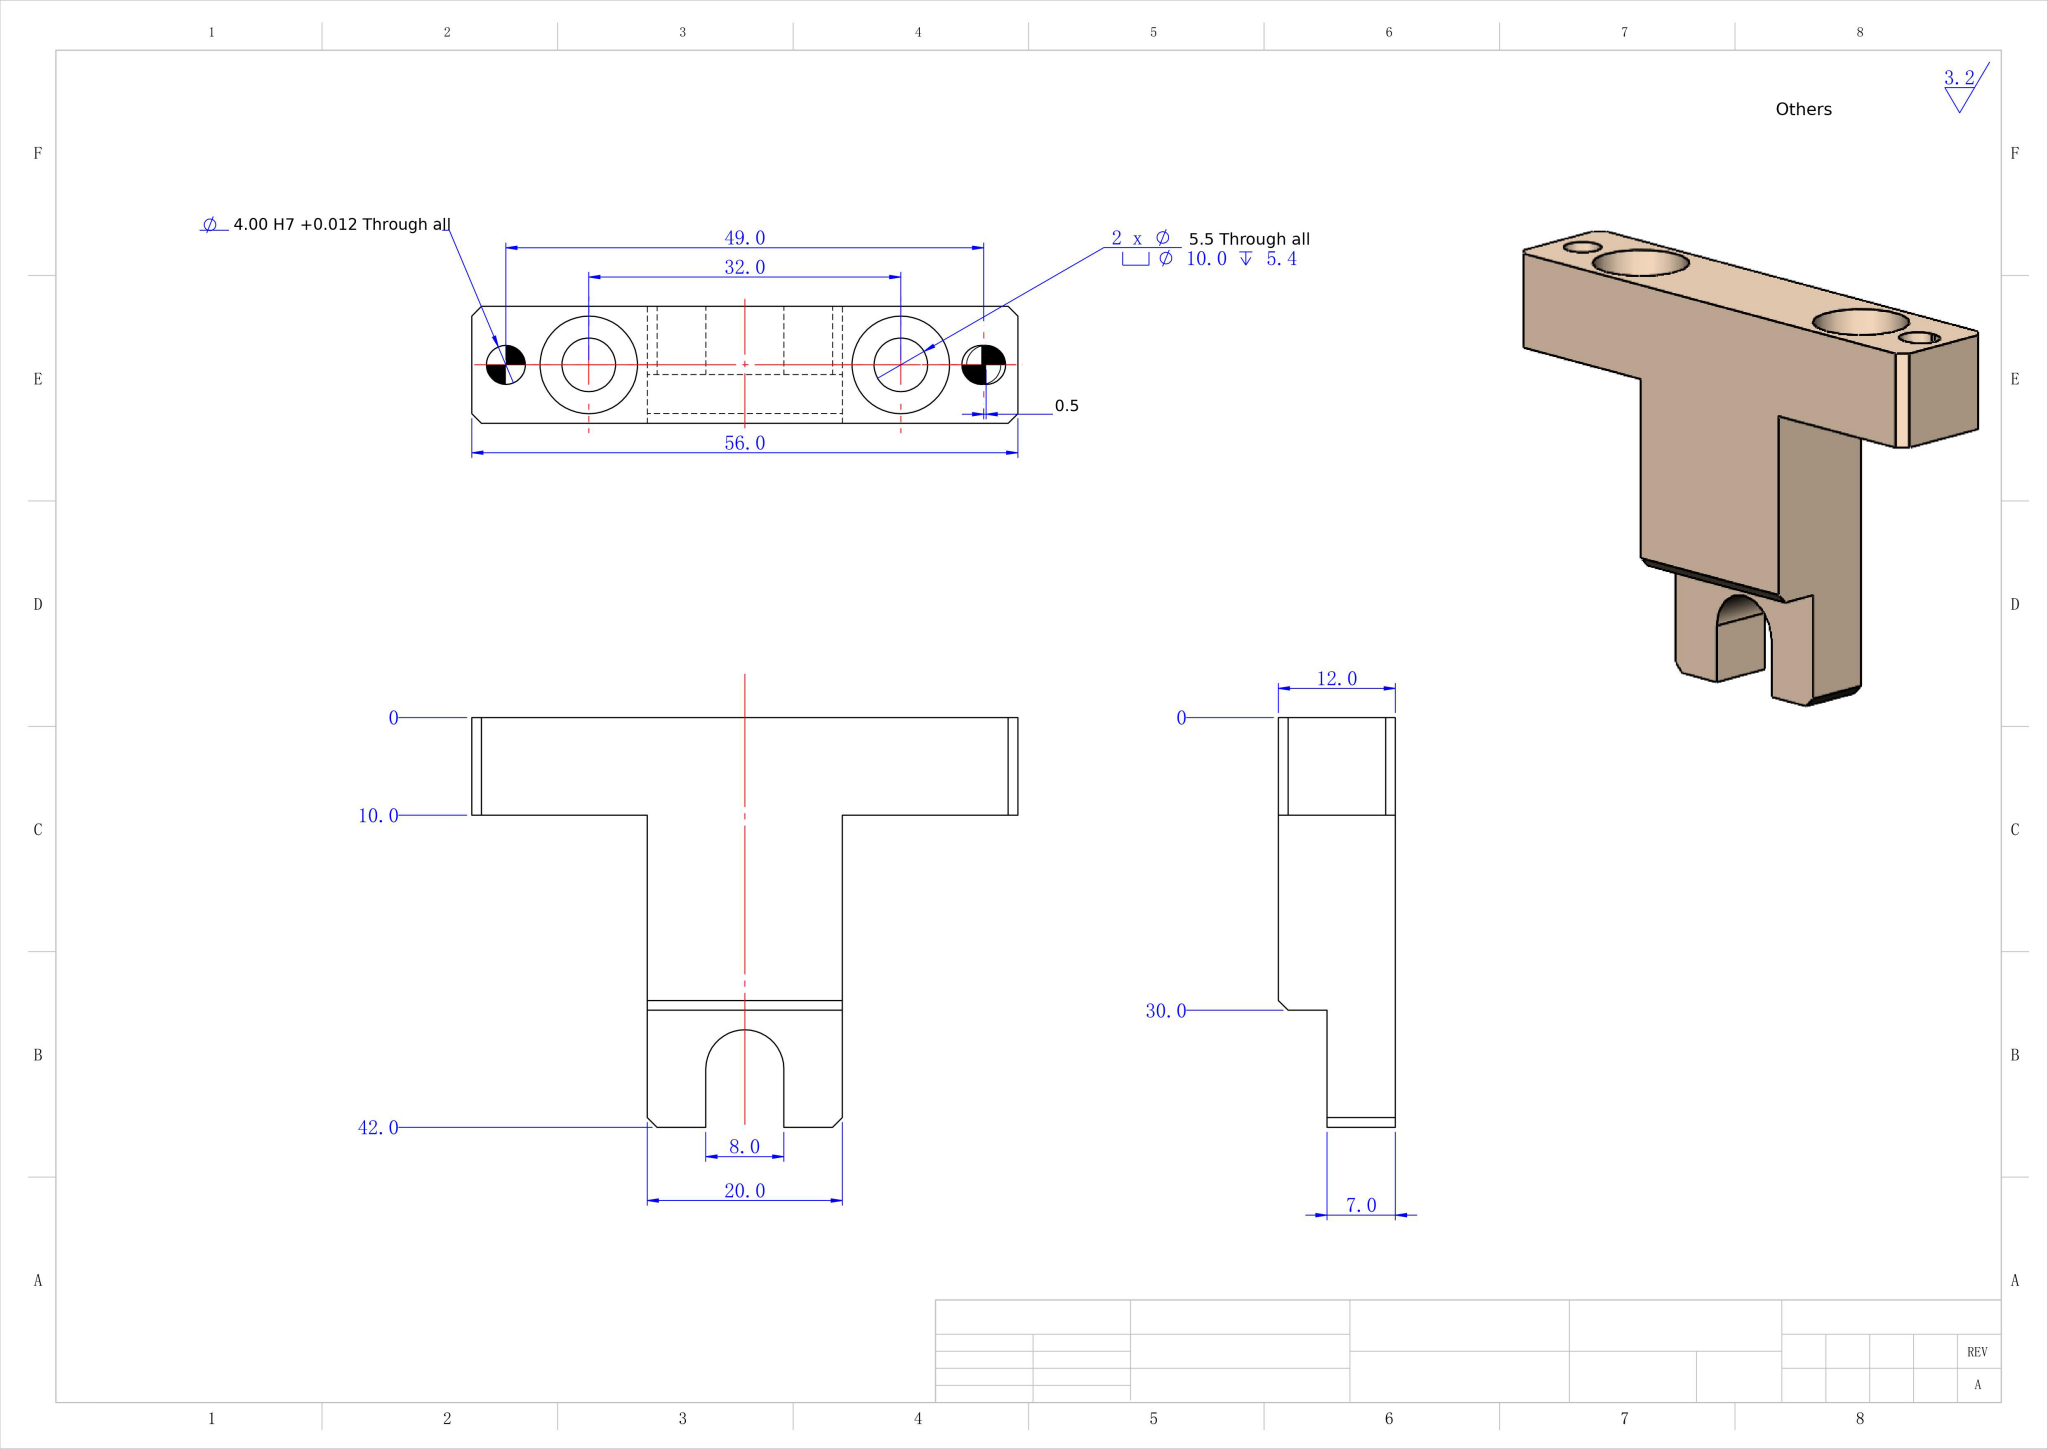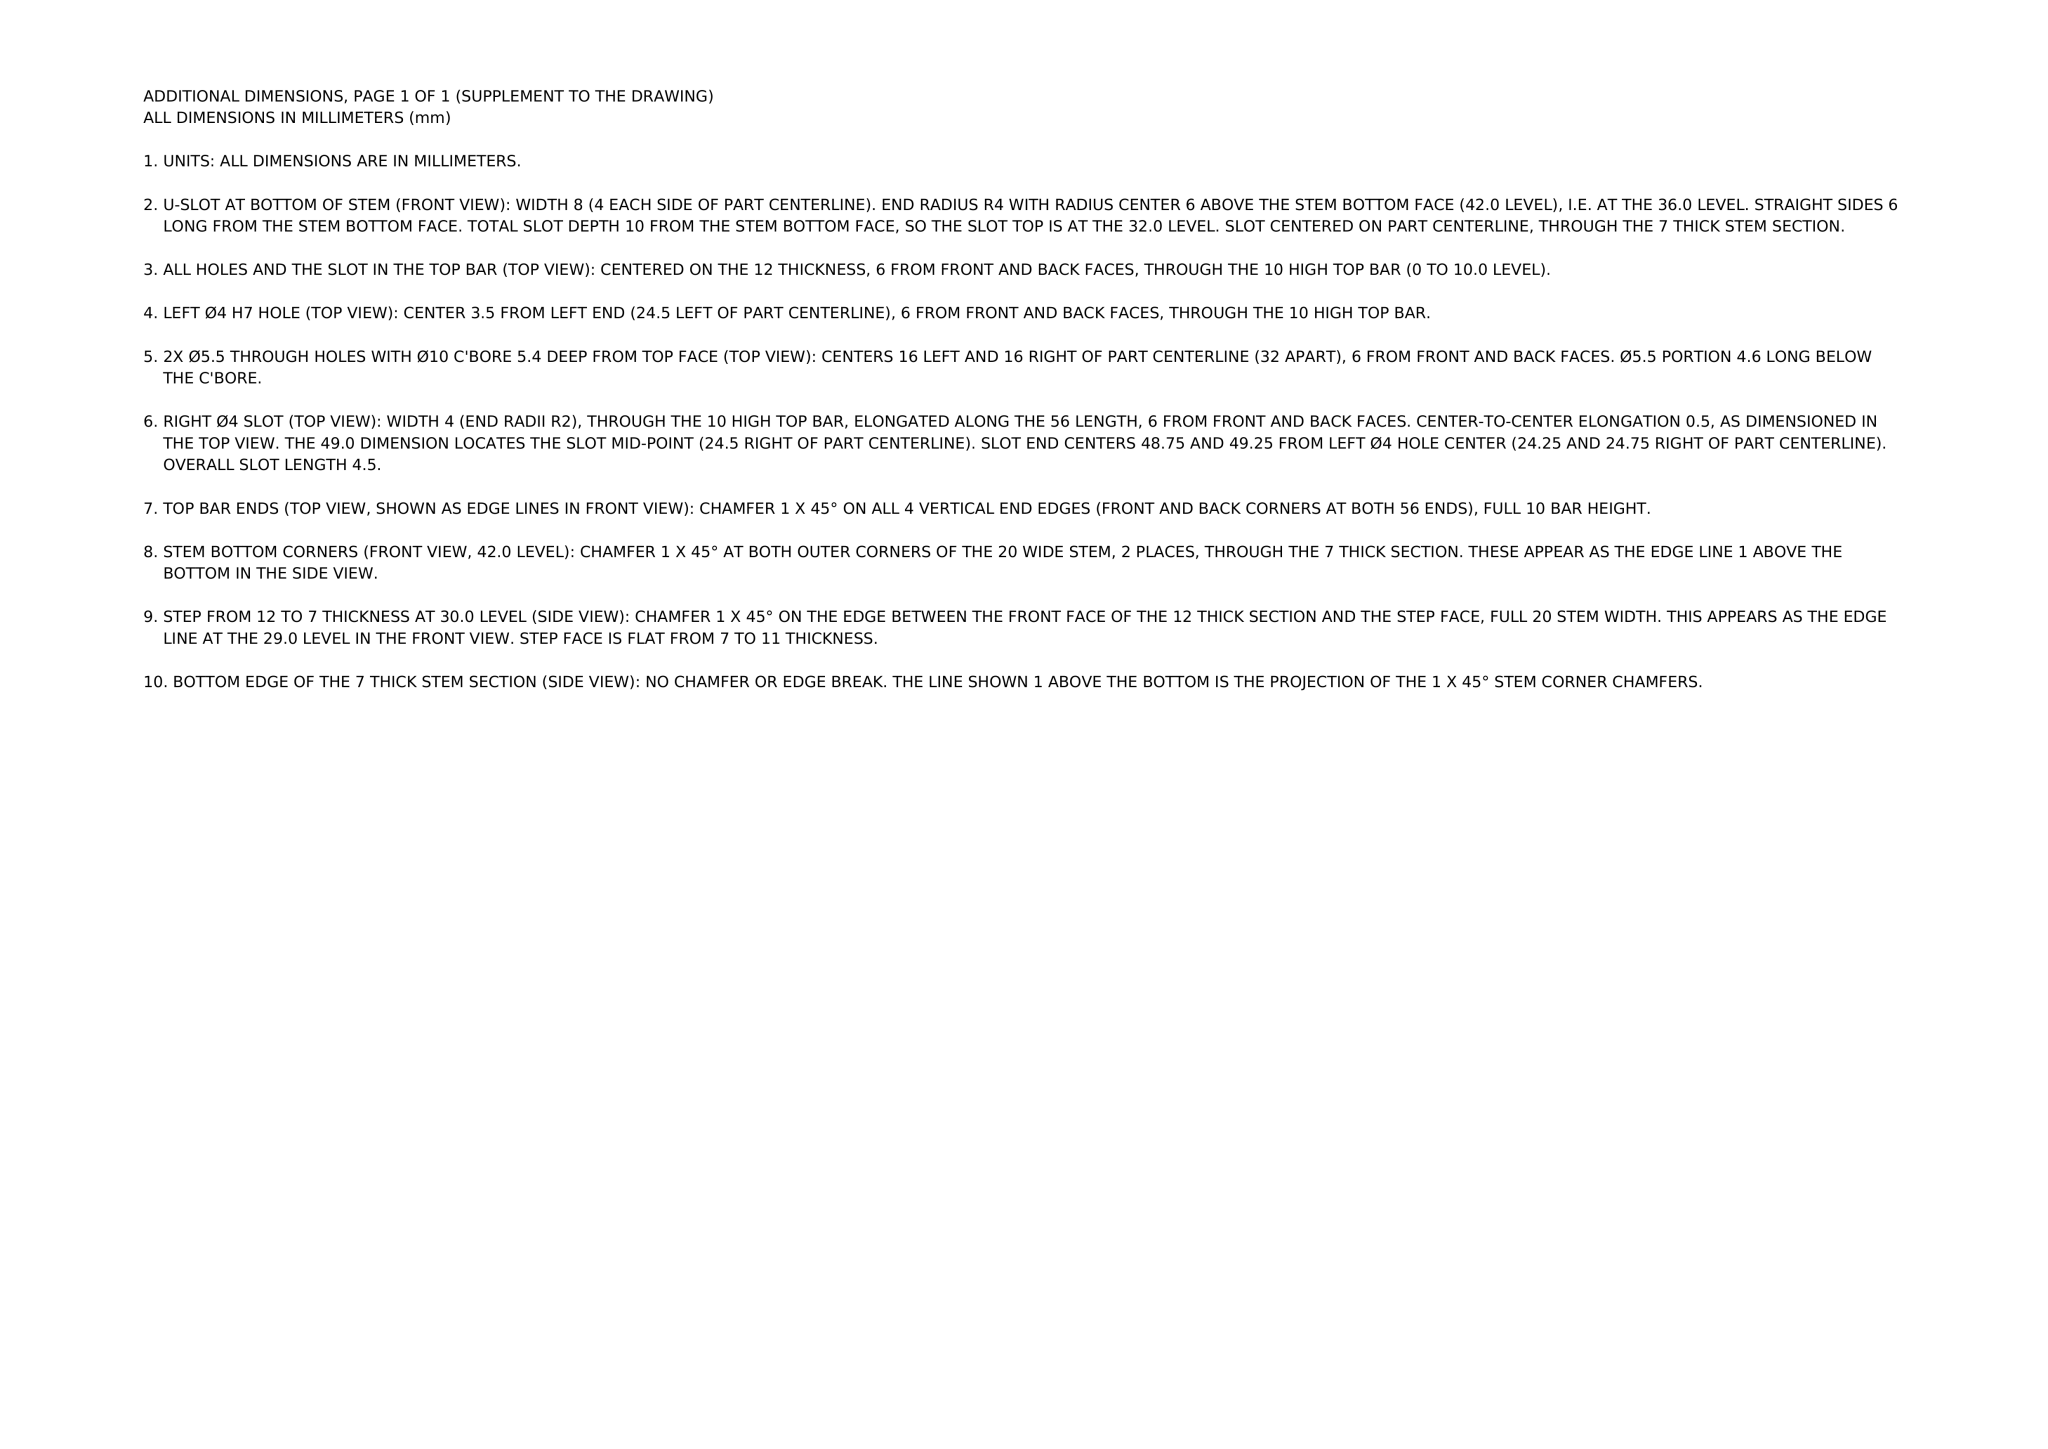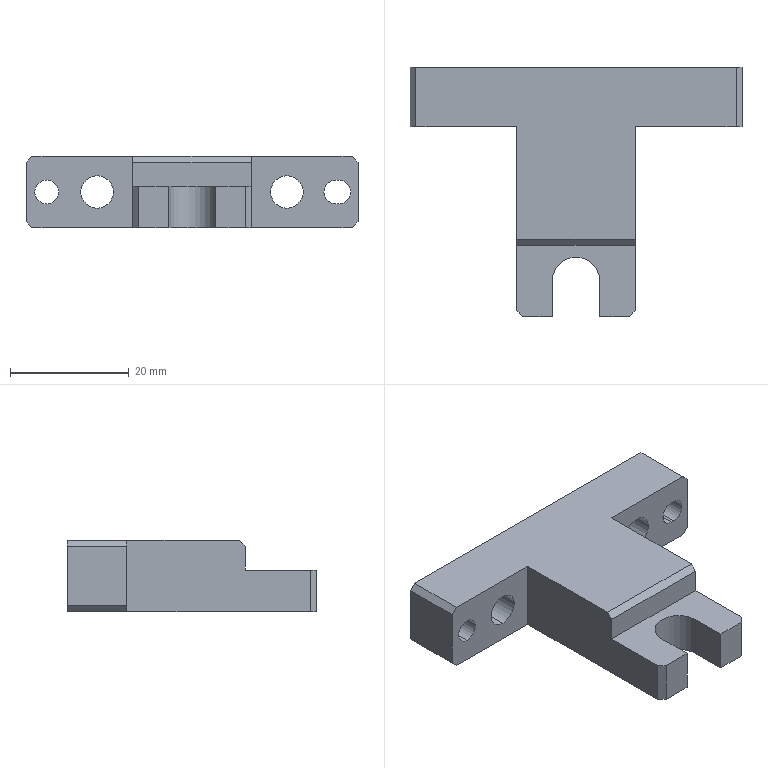Part | NX | mm | 1 solid | 40 faces | box 56 x 42 x 12 mm | volume 11313 mm3 | plane 26 | cylinder 14 | commonest cylinder face diameters 4 x5 10 x4 5.5 x4 8 x1